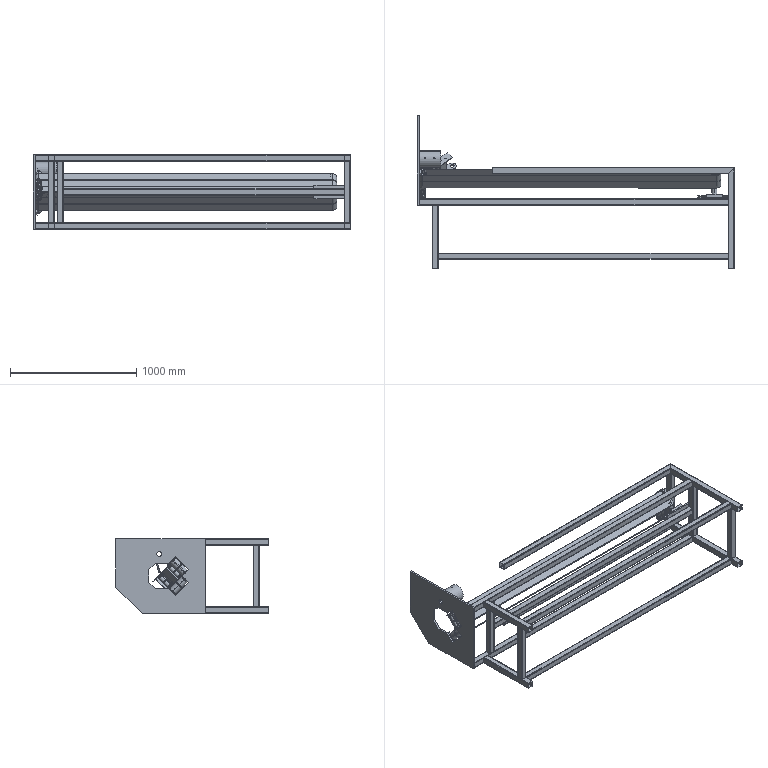Assembly | SolidWorks | mm | 40 component files | 57 solids | 1285 faces | box 2516 x 1210 x 590 mm | volume 21094983 mm3 | cylinder 639 | plane 540 | cone 56 | torus 50 | commonest cylinder face diameters 10 x77 5 x76 3.5 x45 46 x34 28 x28 25 x26 52 x26 11 x24
Bill of materials:
1520F-T | 2 |  | Compact rectangular block body with shafts sticking out of it. One straight round shaft passes through the block and sticks out on both sides. A second short round shaft stub comes out of an adjacent face, perpendicular to the first, from a raised semicircular boss. One face carries a square plate with four small holes near its corners. The shaft ends have small cross holes.
16PlateModified | 1 |  | Thin flat plate, mostly rectangular, with one large angled (chamfered) corner. It has an irregular polygonal cutout with stepped, notched edges and one small round hole above the cutout.
6203 | 2 |  | Thick annular ring (short hollow cylinder) with a plain through-bore and flat end faces. Each face has two thin concentric circular lines, one near the outer edge and one near the bore. Outer edges look slightly rounded. The bore is fairly small compared with the outer diameter, so the ring wall is wide.
BearingHousing6203 | 2 |  | Short hollow cylindrical ring joined along one side to a flat rectangular flange bar. The bar extends past the ring at both ends, and each end has a round through hole. The ring bore appears to have an internal step (counterbore or shoulder).
DriveRoller | 2 |  | Stepped cylinder made of two larger coaxial cylindrical sections separated by a narrow groove. One end has a smaller two-step pin. The other end has a recessed face with a central small hole and a small notch next to it.
InnerHole15b=5SynchronousWheel | 1 |  | Cylindrical toothed wheel with many evenly spaced axial teeth around its circumference and a thin flange at each end. The central round bore has a single rectangular keyway.
Belt | 2 |  | Long, slender straight rod. Both ends appear to have short end sections that are shaded differently and have rounded edges.
Frame | 1 |  | Open rectangular box frame made of straight square-section members: long rails, vertical posts, and cross members. Intermediate rails and posts are included, and some rail ends stick out past the corners. One upper rail is offset and shorter than the full length.
Bearing6205 | 4 |  | Thick annular ring (short hollow cylinder) with a plain through-bore and flat end faces. Each face has two thin concentric circular lines, one near the outer edge and one near the bore. Outer edges look slightly rounded. Similar to unnamed part, but the bore is larger compared with the outer diameter, so the ring wall is narrower.
DovetailPlate | 1 |  | Flat rectangular bar with a dovetail-profile rail running along one face over its full length.
DovetailSlot | 1 |  | Rectangular block with a dovetail-shaped groove profile on one side, joined by a short cylindrical neck to a thin plate that is triangular (pointed) in side view. A curved opening is visible on the narrow top face of the block.
NylonCover | 2 | A-Glass Fiber | Shallow circular disc or cap with a flat solid top face and a stepped outside edge (two diameters). The underside is recessed, leaving an outer annular wall, and has a smaller central circular recess or bore.
StainlessSteelRoller | 2 |  | Thin-walled hollow tube made of two coaxial cylindrical sleeve sections separated by a narrow circumferential groove or step. Both ends are open, and an inner step or ring is visible inside.
SupportRollerAxis | 2 |  | Long solid-looking cylindrical rod with a short larger-diameter collar near one end, followed by a slightly smaller end section. The opposite end face has a small central axial hole.
AdjustingRollerLowerPlate | 1 |  | Straight rectangular bar or flat link with two round through-holes, one near each end.
AdjustingRollerUpperPlate | 1 |  | Straight rectangular bar or flat link with two round through-holes, one near each end.
AdjustingRoundSteel | 1 |  | Solid round rod with one smooth bend into two straight legs. The longer leg has a flat or stepped section along most of its length.
AdjustingWheelEar | 2 |  | Flat plate tab with one full-radius rounded end, a square opposite end, and one round through-hole near the rounded end.
AdjustingWheelPivot | 2 |  | Plain solid cylinder (round bar or pin) with flat ends.
VegetablePressSmallAxis | 3 |  | Stepped cylindrical shaft or pin: a long main diameter with a short reduced-diameter section at each end, and a small axial bore in the end faces.
VegetablePressSmallAxisSleeve | 3 |  | Cylindrical sleeve or bushing with an external circumferential groove part-way along its length, and a stepped (counterbored) internal bore at the ends.
VegetablePressSide | 1 |  | Formed bracket: two parallel profiled side plates joined by a bent web, forming a U or channel shape. The side plates have mounting holes, a lobe with a larger hole, and a tab with a medium hole.
StainlessSteelSleeve_CastIron | 1 |  | Thin-walled round tube section with several small radial through-holes in the wall.
Mates:
1. coincident | Frame-1 face at (2350, 500, 520) dir (0, -1, 0) | AssemblyDriveAxis-1/16PlateModified-1 face at (-125, 500, 565) dir (0, -1, 0)
2. coincident | Frame-1 face at (2350, 545, 565) dir (0, 0, 1) | AssemblyDriveAxis-1/16PlateModified-1 face at (-125, 1210, 565) dir (0, 0, 1)
3. coincident | Frame-1 face at (-125, 545, 560) dir (-1, 0, 0) | AssemblyDriveAxis-1/16PlateModified-1 face at (-125, 500, 565) dir (1, 0, 0)
4. concentric | AssemblyDriveAxis-1/16PlateModified-1 face at (-141, 865, 445) dir (1, 0, 0) r 20 | StainlessSteelSleeve_CastIron-1 face at (45, 865, 445) dir (1, 0, 0) r 56.5
5. coincident | AssemblyDriveAxis-1/16PlateModified-1 face at (-125, 500, 565) dir (1, 0, 0) | StainlessSteelSleeve_CastIron-1 face at (-125, 843.426, 497.219) dir (-1, 0, 0)
6. coincident | Frame-1 face at (2350, 550, 250) dir (0, 1, 0) | PassiveRollerAssembly-1/DovetailPlate-1 face at (2325, 550, 325) dir (0, -1, 0)
7. coincident | Frame-1 face at (2325, 525, 270) dir (1, 0, 0) | PassiveRollerAssembly-1/DovetailPlate-1 face at (2325, 550, 270) dir (1, 0, 0)
8. coincident | Frame-1 edge at (2325, 550, 270) dir (1, 0, 0) | PassiveRollerAssembly-1/DovetailPlate-1 edge at (2325, 550, 270) dir (1, 0, 0)
9. concentric | AssemblyDriveAxis-1/DriveRoller-1 face at (-102, 782.054, 414.962) dir (0, 0.7071, 0.7071) r 29.5 | Belt-2 face at (-102, 758.72, 391.628) dir (0, -0.7071, -0.7071) r 30
10. concentric | AssemblyDriveAxis-1/DriveRoller-2 face at (-102, 782.057, 125.043) dir (0, 0.7071, -0.7071) r 29.5 | Belt-1 face at (-102, 659.728, 247.372) dir (0, 0.7071, -0.7071) r 30
11. tangent | PassiveRollerAssembly-1/StainlessSteelRoller-1 face at (2216.026, 584.48, 218.093) dir (0, -0.7071, -0.7071) r 30 | Belt-2 face at (-101.994, 779.933, 370.415) dir (-0.000215, -0.7071, 0.7071)
12. tangent | PassiveRollerAssembly-1/StainlessSteelRoller-2 face at (2216.026, 584.48, 320.907) dir (0, -0.7071, 0.7071) r 30 | Belt-1 face at (2232.984, 637.652, 225.296) dir (0.0005225, 0.7071, 0.7071)
13. coincident | AssemblyDriveAxis-1/16PlateModified-1 face at (-125, 500, 565) dir (1, 0, 0) | 1520F-T-1 face at (-125, 574.797, 325.829) dir (-1, 0, 0)
14. parallel | AssemblyDriveAxis-1/1520F-T-1 face at (-125, 594.668, 270.003) dir (0, -0.7071, -0.7071) | 1520F-T-1 face at (-79, 574.795, 283.401) dir (0, -0.7071, -0.7071)
15. distance | Belt-1 face at (-101.984, 682.001, 269.646) dir (0.0005225, 0.7071, 0.7071) | SmallAxisAssembly-1/VegetablePressSide-1 face at (-4.446, 759.835, 194.569) dir (-0.0005225, -0.7071, -0.7071)
16. distance | SmallAxisAssembly-1/VegetablePressSmallAxisSleeve-1 face at (-106.324, 707.292, 268.075) dir (-0.0005225, -0.7071, -0.7071) r 17.5 | Belt-2 face at (-102, 758.72, 391.628) dir (0, -0.7071, -0.7071) r 31.5
17. distance | AssemblyDriveAxis-1/DriveRoller-1 face at (-92.499, 761.632, 390.129) dir (0, 0.7071, 0.7071) | Belt-2 face at (-102, 758.72, 391.628) dir (0, 0.7071, 0.7071)
18. distance | AssemblyDriveAxis-1/DriveRoller-2 face at (-92, 759.479, 147.72) dir (0, 0.7071, -0.7071) | Belt-1 face at (-102, 758.722, 148.377) dir (0, 0.7071, -0.7071)
19. concentric | 1520F-T-1 face at (-59.49, -110.1, 17.253) dir (1, 0, 0) r 7.5 | DriveRoller-1 face at (-218.215, -110.1, 17.253) dir (-1, 0, 0) r 8.5
20. coincident | 1520F-T-1 face at (-77.715, -110.1, 17.253) dir (-1, 0, 0) | DriveRoller-1 face at (-77.715, -102.974, 14.914) dir (1, 0, 0)
21. concentric | 1520F-T-1 face at (-13.213, -110.1, -48.978) dir (0, 0, 1) r 7.5 | DriveRoller-2 face at (-13.213, -110.1, -187.753) dir (0, 0, -1) r 29.5
22. coincident | 1520F-T-1 face at (-13.213, -110.1, -47.253) dir (0, 0, -1) | DriveRoller-2 face at (-13.265, -102.6, -47.253) dir (0, 0, 1)
23. concentric | 1520F-T-1 face at (-59.49, -110.1, 17.253) dir (1, 0, 0) r 7.5 | InnerHole15b=5SynchronousWheel-1 face at (-17.701, -110.1, 17.253) dir (-1, 0, 0) r 7.5
24. distance | 1520F-T-1 face at (51.289, -110.1, 17.253) dir (1, 0, 0) | InnerHole15b=5SynchronousWheel-1 face at (59.289, -102.6, 17.253) dir (1, 0, 0)
25. coincident | 1520F-T-1 face at (-13.213, -133.1, 17.253) dir (0, -1, 0) | 16PlateModified-1 face at (-124.865, -133.1, 322.788) dir (0, 1, 0)
26. coincident | 1520F-T-1 face at (16.789, -133.1, -12.751) dir (0, 0, -1) | 16PlateModified-1 face at (-124.865, -149.1, -12.751) dir (0, 0, -1)
27. coincident | 1520F-T-1 face at (-43.211, -133.1, -12.751) dir (-1, 0, 0) | 16PlateModified-1 face at (-43.211, -149.1, 322.788) dir (-1, 0, 0)
28. concentric | DriveRoller-1 face at (-218.215, -110.1, 17.253) dir (-1, 0, 0) r 8.5 | 6203-1 face at (-206.215, -110.1, 17.253) dir (-1, 0, 0) r 20
29. coincident | DriveRoller-1 face at (-206.215, -102.024, 14.602) dir (-1, 0, 0) | 6203-1 face at (-206.215, -101, 17.253) dir (1, 0, 0)
30. concentric | 6203-1 face at (-206.215, -110.1, 17.253) dir (-1, 0, 0) r 20 | BearingHousing6203-1 face at (-178.487, -110.1, 17.253) dir (1, 0, 0) r 20
31. coincident | 6203-1 face at (-218.215, -98.6, 17.253) dir (-1, 0, 0) | BearingHousing6203-1 face at (-218.215, -90.1, 17.253) dir (1, 0, 0)
32. concentric | DriveRoller-2 face at (-13.213, -110.1, -187.753) dir (0, 0, -1) r 8.5 | 6203-2 face at (-13.213, -110.1, -187.753) dir (0, 0, 1) r 20
33. coincident | DriveRoller-2 face at (-13.272, -101.6, -175.753) dir (0, 0, -1) | 6203-2 face at (-9.98, -99.064, -175.753) dir (0, 0, 1)
34. concentric | 6203-2 face at (-13.213, -110.1, -187.753) dir (0, 0, 1) r 20 | BearingHousing6203-2 face at (-13.213, -110.1, -148.026) dir (0, 0, 1) r 20
35. coincident | 6203-2 face at (-10.655, -101.367, -187.753) dir (0, 0, -1) | BearingHousing6203-2 face at (-13.213, -90.1, -187.753) dir (0, 0, 1)
36. coincident | 16PlateModified-1 face at (-124.865, -133.1, 322.788) dir (0, 1, 0) | BearingHousing6203-1 face at (-227.715, -133.1, -27.747) dir (0, -1, 0)
37. coincident | 16PlateModified-1 face at (-124.865, -133.1, 322.788) dir (0, 1, 0) | BearingHousing6203-2 face at (31.787, -133.1, -197.253) dir (0, -1, 0)
38. coincident | DovetailPlate-1 face at (-59.177, 0.2062, 360) dir (0, 1, 0) | DovetailSlot-1 face at (-58.677, 0.2062, 311.026) dir (0, -1, 0)
39. coincident | DovetailPlate-1 face at (-24.677, 0.2062, 360) dir (-0.6196, -0.7849, 0) | DovetailSlot-1 face at (-24.677, 0.2062, 311.026) dir (0.6196, 0.7849, 0)
40. coincident | DovetailSlot-1 face at (-12.834, 83.25, 251.026) dir (-0.7071, 0.7071, 0) | SupportRollerAxis-1 face at (-12.834, 83.25, 251.026) dir (0.7071, -0.7071, 0)
41. concentric | DovetailSlot-1 face at (-12.834, 83.25, 251.026) dir (-0.7071, 0.7071, 0) r 12.5 | SupportRollerAxis-1 face at (41.829, 28.587, 251.026) dir (0.7071, -0.7071, 0) r 12.5
42. concentric | Bearing6205-1 face at (-43.947, 114.363, 251.026) dir (0.7071, -0.7071, 0) r 12.5 | SupportRollerAxis-1 face at (41.829, 28.587, 251.026) dir (0.7071, -0.7071, 0) r 12.5
43. coincident | Bearing6205-1 face at (-23.894, 113.203, 260.278) dir (0.7071, -0.7071, 0) | SupportRollerAxis-1 face at (-41.067, 96.03, 242.274) dir (-0.7071, 0.7071, 0)
44. concentric | SupportRollerAxis-1 face at (41.829, 28.587, 251.026) dir (0.7071, -0.7071, 0) r 12.5 | Bearing6205-3 face at (-104.758, 175.174, 251.026) dir (-0.7071, 0.7071, 0) r 12.5
45. coincident | SupportRollerAxis-1 face at (-122.263, 178.882, 243.212) dir (-0.7071, 0.7071, 0) | Bearing6205-3 face at (-103.874, 197.271, 251.026) dir (-0.7071, 0.7071, 0)
46. concentric | DovetailSlot-1 face at (5.48, 83.25, 251.026) dir (0.7071, 0.7071, 0) r 12.5 | SupportRollerAxis-2 face at (-49.183, 28.587, 251.026) dir (-0.7071, -0.7071, 0) r 12.5
47. coincident | DovetailSlot-1 face at (5.48, 83.25, 251.026) dir (0.7071, 0.7071, 0) | SupportRollerAxis-2 face at (5.48, 83.25, 251.026) dir (-0.7071, -0.7071, 0)
48. concentric | Bearing6205-2 face at (25.986, 103.756, 251.026) dir (0.7071, 0.7071, 0) r 12.5 | SupportRollerAxis-2 face at (-49.183, 28.587, 251.026) dir (-0.7071, -0.7071, 0) r 12.5
49. coincident | Bearing6205-2 face at (17.921, 111.821, 258.249) dir (-0.7071, -0.7071, 0) | SupportRollerAxis-2 face at (16.939, 112.803, 245.342) dir (0.7071, 0.7071, 0)
50. concentric | SupportRollerAxis-2 face at (-49.183, 28.587, 251.026) dir (-0.7071, -0.7071, 0) r 12.5 | Bearing6205-4 face at (108.01, 185.781, 251.026) dir (-0.7071, -0.7071, 0) r 12.5
51. coincident | SupportRollerAxis-2 face at (99.933, 193.858, 245.951) dir (0.7071, 0.7071, 0) | Bearing6205-4 face at (107.83, 185.961, 237.529) dir (0.7071, 0.7071, 0)
52. coincident | Bearing6205-2 face at (26.885, 124.071, 259.72) dir (0.7071, 0.7071, 0) | StainlessSteelRoller-2 face at (22.45, 128.505, 251.026) dir (-0.7071, -0.7071, 0)
53. concentric | Bearing6205-2 face at (25.986, 103.756, 251.026) dir (0.7071, 0.7071, 0) r 26 | StainlessSteelRoller-2 face at (-55.084, 22.686, 251.026) dir (-0.7071, -0.7071, 0) r 30
54. coincident | Bearing6205-1 face at (-36.099, 122.211, 258.712) dir (-0.7071, 0.7071, 0) | StainlessSteelRoller-1 face at (-54.985, 103.325, 238.523) dir (0.7071, -0.7071, 0)
55. concentric | Bearing6205-1 face at (-43.947, 114.363, 251.026) dir (0.7071, -0.7071, 0) r 26 | StainlessSteelRoller-1 face at (47.73, 22.686, 251.026) dir (0.7071, -0.7071, 0) r 30
56. concentric | StainlessSteelRoller-1 face at (47.73, 22.686, 251.026) dir (0.7071, -0.7071, 0) r 30 | NylonCover-1 face at (-132.335, 202.751, 251.026) dir (-0.7071, 0.7071, 0) r 30
57. coincident | StainlessSteelRoller-1 face at (-143.235, 180.537, 232.271) dir (-0.7071, 0.7071, 0) | NylonCover-1 face at (-109.768, 214.005, 232.913) dir (0.7071, -0.7071, 0)
58. concentric | StainlessSteelRoller-2 face at (-55.084, 22.686, 251.026) dir (-0.7071, -0.7071, 0) r 30 | NylonCover-2 face at (124.981, 202.751, 251.026) dir (0.7071, 0.7071, 0) r 30
59. coincident | StainlessSteelRoller-2 face at (98.111, 218.308, 251.026) dir (0.7071, 0.7071, 0) | NylonCover-2 face at (139.136, 177.283, 240.302) dir (-0.7071, -0.7071, 0)
60. concentric | VegetablePressSmallAxisSleeve-1 face at (-52.23, 0, 0) dir (-1, 0, 0) r 8 | VegetablePressSmallAxis-1 face at (63, 0, 0) dir (1, 0, 0) r 6
61. coincident | VegetablePressSmallAxisSleeve-1 face at (-48, 8, 0) dir (-1, 0, 0) | VegetablePressSmallAxis-1 face at (-48, 6, 0) dir (-1, 0, 0)
62. concentric | VegetablePressSmallAxis-1 face at (63, 0, 0) dir (1, 0, 0) r 6 | VegetablePressSide-1 face at (-63, 0, 0) dir (-1, 0, 0) r 3
63. concentric | VegetablePressSide-1 face at (-67.001, 132.208, 13.668) dir (1, 0, 0) r 3 | SmallAxisAssembly1-1/VegetablePressSmallAxis-1 face at (63, 132.208, 13.668) dir (1, 0, 0) r 6
64. coincident | VegetablePressSmallAxis-1 edge at (-63, 0, 0) dir (1, 0, 0) r 6 | VegetablePressSide-1 face at (-63, 113.912, 73.138) dir (1, 0, 0)
65. coincident | VegetablePressSide-1 face at (-63, 113.912, 73.138) dir (1, 0, 0) | SmallAxisAssembly1-1/VegetablePressSmallAxis-1 face at (-63, 132.208, 13.668) dir (-1, 0, 0)
66. concentric | VegetablePressSide-1 face at (67, 120.691, 71.125) dir (-1, 0, 0) r 6 | AdjustingRoundSteel-1 face at (-67, 120.691, 71.125) dir (1, 0, 0) r 6
67. coincident | VegetablePressSide-1 face at (-67, 113.912, 73.138) dir (-1, 0, 0) | AdjustingRoundSteel-1 face at (-67, 120.691, 71.125) dir (-1, 0, 0)
68. coincident | AdjustingRollerLowerPlate-1 face at (62, 117.599, 65.172) dir (0, 0.8091, 0.5876) | AdjustingRoundSteel-1 face at (-67, 115.836, 67.6) dir (0, -0.8091, -0.5876)
69. coincident | AdjustingRollerLowerPlate-1 face at (0, 104.806, 65.769) dir (0, -0.5876, 0.8091) | AdjustingRoundSteel-1 face at (61.068, 117.752, 75.171) dir (0, -0.5876, 0.8091)
70. distance | VegetablePressSide-1 edge at (63, 109.516, 70.754) dir (0, 0.4766, -0.8791) | AdjustingRollerLowerPlate-1 face at (62, 101.416, 53.42) dir (1, 0, 0)
71. concentric | AdjustingRollerLowerPlate-1 face at (47, 109.507, 59.296) dir (0, -0.5876, 0.8091) r 5.5 | AdjustingWheelPivot-1 face at (47, 109.507, 59.296) dir (0, -0.5876, 0.8091) r 5
72. concentric | AdjustingRollerLowerPlate-1 face at (-47, 109.507, 59.296) dir (0, -0.5876, 0.8091) r 5.5 | AdjustingWheelPivot-2 face at (-47, 109.507, 59.296) dir (0, -0.5876, 0.8091) r 5
73. coincident | AdjustingRollerLowerPlate-1 face at (0, 109.507, 59.296) dir (0, 0.5876, -0.8091) | AdjustingWheelPivot-1 face at (47, 109.507, 59.296) dir (0, 0.5876, -0.8091)
74. coincident | AdjustingRollerLowerPlate-1 face at (0, 109.507, 59.296) dir (0, 0.5876, -0.8091) | AdjustingWheelPivot-2 face at (-47, 109.507, 59.296) dir (0, 0.5876, -0.8091)
75. concentric | AdjustingWheelPivot-1 face at (47, 109.507, 59.296) dir (0, -0.5876, 0.8091) r 5 | AdjustingRollerUpperPlate-1 face at (47, 91.879, 83.57) dir (0, 0.5876, -0.8091) r 5.5
76. concentric | AdjustingWheelPivot-2 face at (-47, 109.507, 59.296) dir (0, -0.5876, 0.8091) r 5 | AdjustingRollerUpperPlate-1 face at (-47, 91.879, 83.57) dir (0, 0.5876, -0.8091) r 5.5
77. coincident | AdjustingWheelPivot-1 face at (47, 91.879, 83.57) dir (0, -0.5876, 0.8091) | AdjustingRollerUpperPlate-1 face at (0, 91.879, 83.57) dir (0, -0.5876, 0.8091)
78. coincident | AdjustingRollerUpperPlate-1 face at (63, 83.787, 77.694) dir (1, 0, 0) | AdjustingWheelEar-1 face at (63, 71.312, 111.89) dir (-1, 0, 0)
79. coincident | AdjustingRollerUpperPlate-1 face at (0, 96.58, 77.097) dir (0, 0.5876, -0.8091) | AdjustingWheelEar-1 face at (63, 88.488, 71.221) dir (0, 0.5876, -0.8091)
80. coincident | AdjustingRollerUpperPlate-1 face at (-63, 83.787, 77.694) dir (0, -0.8091, -0.5876) | AdjustingWheelEar-1 face at (63, 63.221, 106.014) dir (0, -0.8091, -0.5876)
81. coincident | AdjustingRollerUpperPlate-1 face at (-63, 83.787, 77.694) dir (-1, 0, 0) | AdjustingWheelEar-2 face at (-63, 71.312, 111.89) dir (1, 0, 0)
82. coincident | AdjustingRollerUpperPlate-1 face at (0, 96.58, 77.097) dir (0, 0.5876, -0.8091) | AdjustingWheelEar-2 face at (-66, 88.488, 71.221) dir (0, 0.5876, -0.8091)
83. coincident | AdjustingRollerUpperPlate-1 face at (-63, 83.787, 77.694) dir (0, -0.8091, -0.5876) | AdjustingWheelEar-2 face at (-66, 63.221, 106.014) dir (0, -0.8091, -0.5876)
84. concentric | AdjustingWheelEar-2 edge at (-63, 80.126, 99.753) dir (-1, 0, 0) r 3.5 | SmallAxisAssembly1-2/VegetablePressSmallAxis-1 face at (63, 80.126, 99.753) dir (1, 0, 0) r 6
85. coincident | AdjustingWheelEar-2 face at (-63, 71.312, 111.89) dir (1, 0, 0) | SmallAxisAssembly1-2/VegetablePressSmallAxis-1 face at (-63, 80.126, 99.753) dir (-1, 0, 0)
86. concentric | VegetablePressSmallAxisSleeve-1 face at (-52.23, 0, 0) dir (-1, 0, 0) r 8 | VegetablePressSmallAxis-1 face at (63, 0, 0) dir (1, 0, 0) r 6
87. coincident | VegetablePressSmallAxisSleeve-1 face at (-48, 8, 0) dir (-1, 0, 0) | VegetablePressSmallAxis-1 face at (-48, 6, 0) dir (-1, 0, 0)